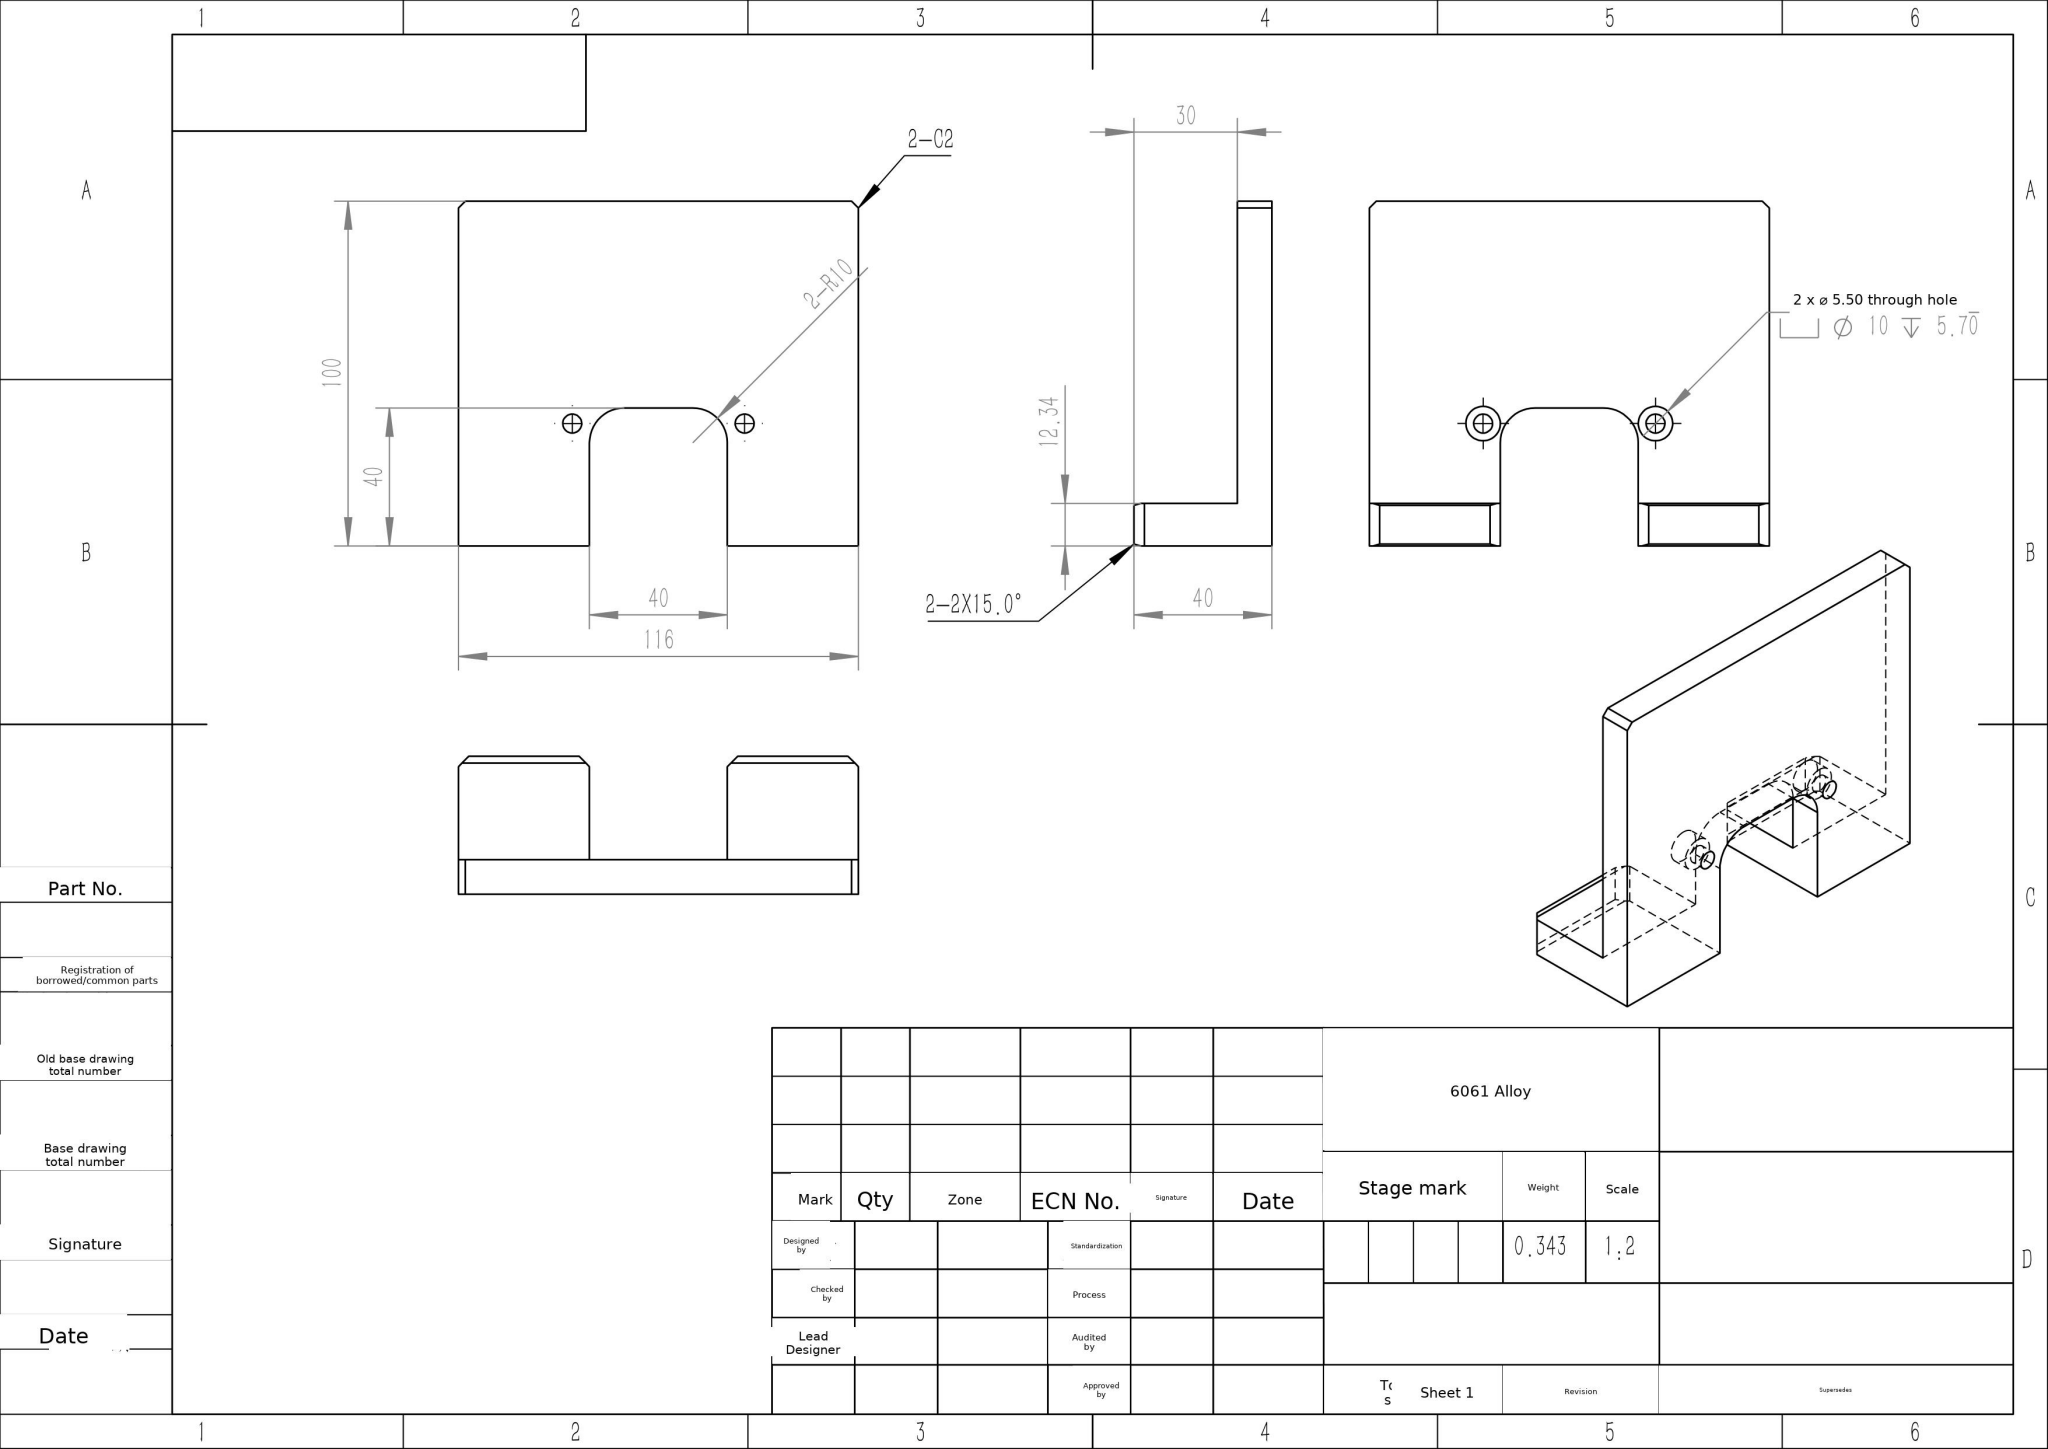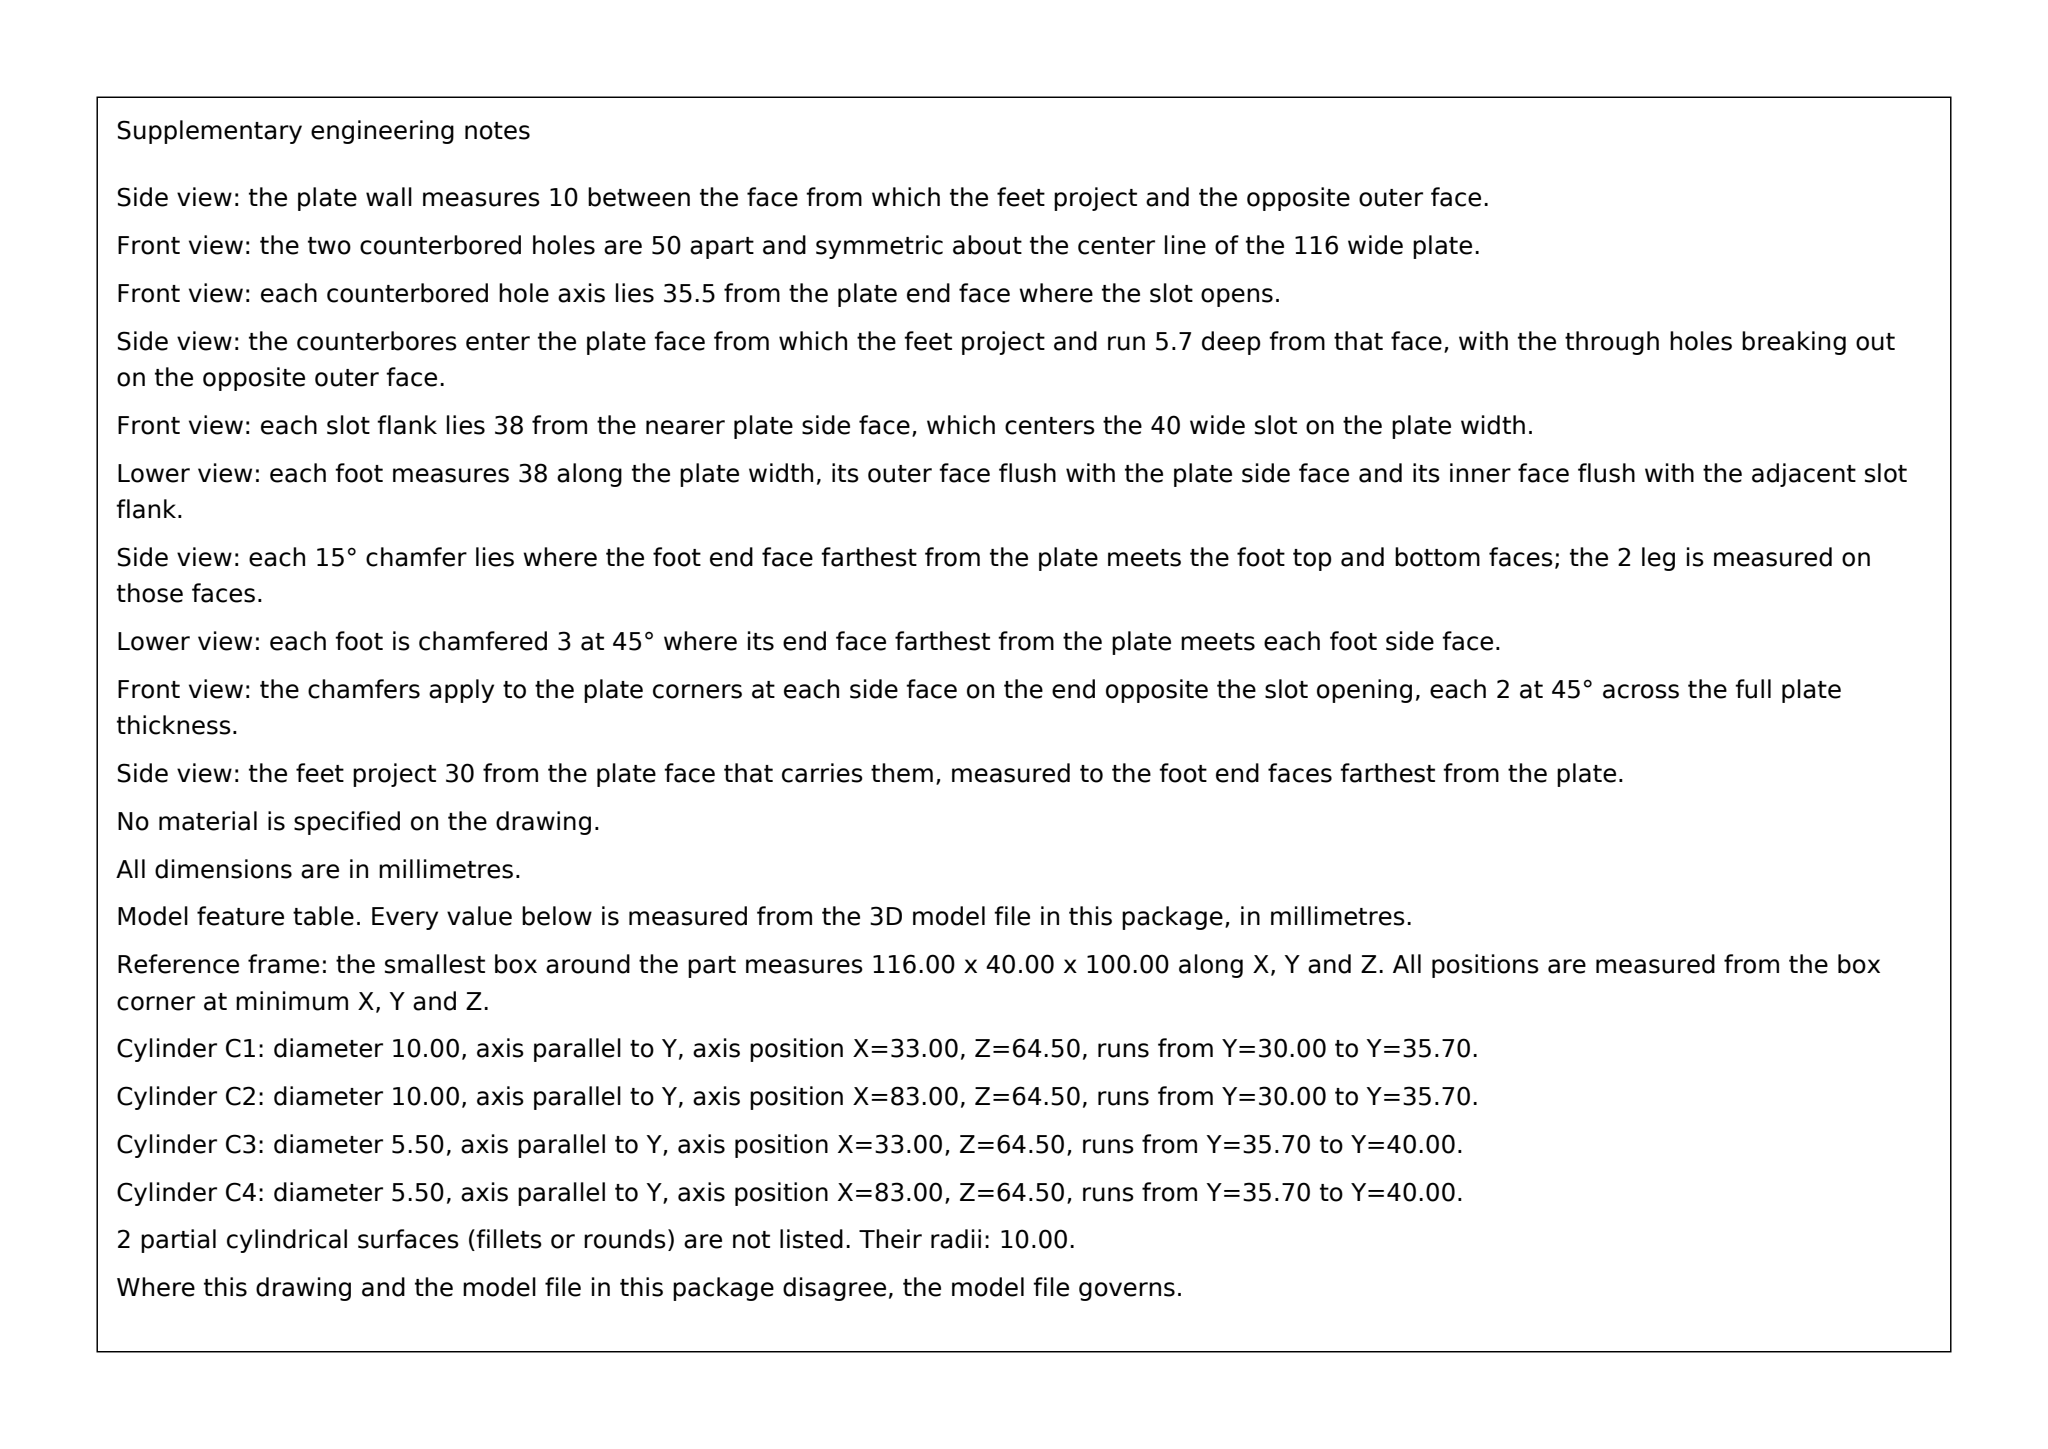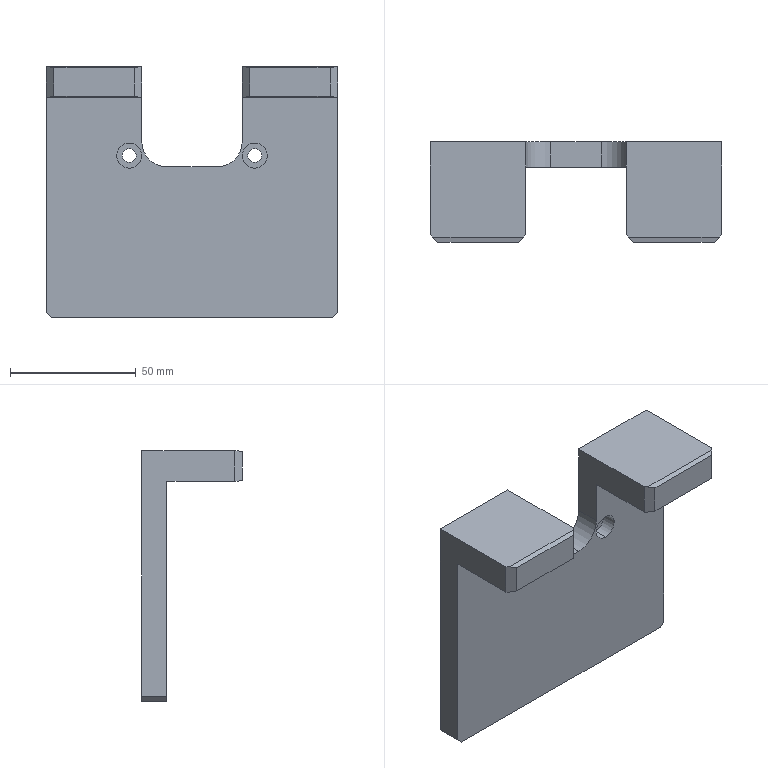Part | SolidWorks | mm | 1 solid | 36 faces | box 116 x 40 x 100 mm | volume 127128 mm3 | plane 26 | cylinder 10 | commonest cylinder face diameters 10 x4 5.5 x4 20 x2
Drawing notes:
2X Ø5.50 CBORE HOLES: 33 & 83 FROM LH EDGE, 50 CTR-CTR | from the solid: cyl dia5.5/dia10 at x=33.0 and x=83.0 (bbox x=116, so symm abt CL; spacing 50)
CBORE HOLE CL 64.5 FROM TOP EDGE (35.5 FROM BOT EDGE) | from the solid: cyl pos z=64.5 of 100 tall bbox; slot top plane z=60 = 40 from bottom
VERT PLATE THK 10 (SIDE VIEW FACES 30 TO 40) | from the solid: y-normal planes at 30.0 and 40.0; bbox y=40
2-2X15.0° CHAMF ON FRONT BOT EDGE OF EA FOOT, BASE THK 12.34 | from the solid: z-planes 87.66 (2X, foot top) vs bbox z=100; chamfer edge at y=0 / z=100
build123d program:
from build123d import *
from OCP.BRepFilletAPI import BRepFilletAPI_MakeChamfer

# Parameters (mm, degrees)
SKETCH1_W                                       = 116
SKETCH1_H                                       = 100
BOSS_EXTRUDE1_DEPTH                             = 10
M5_HEX_SOCKET_HEAD_CAP_SCREW_CBORE1_D           = 5.5
M5_HEX_SOCKET_HEAD_CAP_SCREW_CBORE1_DEPTH       = 10
M5_HEX_SOCKET_HEAD_CAP_SCREW_CBORE1_CBORE_D     = 10
M5_HEX_SOCKET_HEAD_CAP_SCREW_CBORE1_CBORE_DEPTH = 5.7
F_5_0MM_DOWEL_PIN_HOLE1_D                       = 5
F_5_0MM_DOWEL_PIN_HOLE1_DEPTH                   = 10
F_12_0_12_DIAMETER_HOLE1_D                      = 12
CHAMFER1_SIZE                                   = 2
CUT_EXTRUDE2_DEPTH                              = 78.227
SKETCH10_W                                      = 38
SKETCH10_H                                      = 12.339
BOSS_EXTRUDE2_DEPTH                             = 30
CHAMFER2_SIZE                                   = 2
CHAMFER2_SIZE2                                  = 0.5359
CHAMFER3_SIZE                                   = 3


with BuildPart() as part:
    # Sketch1 → Boss-Extrude1 (new body)
    with BuildSketch(Plane(origin=(0, 0, 0), x_dir=(1, 0, 0), z_dir=(0, 1, 0))):
        Rectangle(SKETCH1_W, SKETCH1_H)
    extrude(amount=BOSS_EXTRUDE1_DEPTH)

    # M5 Hex Socket Head Cap Screw CBORE1
    with Locations(Plane(origin=(0, 0, 0), x_dir=(-1, 0, 0), z_dir=(0, -1, 0))):
        with Locations((-25, 55.5), (25, 55.5), (25, -14.5), (-25, -14.5)):
            CounterBoreHole(M5_HEX_SOCKET_HEAD_CAP_SCREW_CBORE1_D / 2, M5_HEX_SOCKET_HEAD_CAP_SCREW_CBORE1_CBORE_D / 2, M5_HEX_SOCKET_HEAD_CAP_SCREW_CBORE1_CBORE_DEPTH, depth=M5_HEX_SOCKET_HEAD_CAP_SCREW_CBORE1_DEPTH)

    # 5.0mm Dowel Pin Hole1
    with Locations(Plane(origin=(0, 0, 0), x_dir=(-1, 0, 0), z_dir=(0, -1, 0))):
        with Locations((15, 55.5), (-15, -14.5)):
            Hole(F_5_0MM_DOWEL_PIN_HOLE1_D / 2, depth=F_5_0MM_DOWEL_PIN_HOLE1_DEPTH)

    # 12.0 _12_ Diameter Hole1 (through all)
    with Locations(Plane(origin=(0, 0, 0), x_dir=(-1, 0, 0), z_dir=(0, -1, 0))):
        with Locations((10, -47.5)):
            Hole(F_12_0_12_DIAMETER_HOLE1_D / 2)

    # Chamfer1
    chamfer1_edges = [part.edges().sort_by_distance(p)[0] for p in [
        (-58, 5, -50),
        (58, 5, -50),
    ]]
    chamfer(chamfer1_edges, length=CHAMFER1_SIZE)

    # Sketch9 → Cut-Extrude2 (cut, through all)
    with BuildSketch(Plane.XZ):
        with BuildLine():
            Line((20, 50), (20, 48))
            Line((20, 48), (20, 20))
            ThreePointArc((20, 20), (17.071, 12.929), (10, 10))
            Line((10, 10), (-10, 10))
            ThreePointArc((-10, 10), (-17.071, 12.929), (-20, 20))
            Line((-20, 20), (-20, 50))
            Line((-20, 50), (20, 50))
        make_face()
    extrude(amount=-CUT_EXTRUDE2_DEPTH, mode=Mode.SUBTRACT)

    # Sketch10 → Boss-Extrude2 (add)
    with BuildSketch(Plane.XZ):
        with Locations((39, 43.831)):
            Rectangle(SKETCH10_W, SKETCH10_H)
        with Locations((-39, 43.831)):
            Rectangle(SKETCH10_W, SKETCH10_H)
    extrude(amount=BOSS_EXTRUDE2_DEPTH)

    # Chamfer2: one chamfer whose edges measure the first distance from different faces: ONE call of the kernel's chamfer builder (chamfer() names one face for all edges)
    chamfer2_edges_1 = [part.edges().sort_by_distance(p)[0] for p in [
        (-39, -30, 37.661),
    ]]
    chamfer2_side_1 = [part.faces().sort_by_distance(p)[0] for p in [
        (-39, -15, 37.661),
    ]]
    chamfer2_edges_2 = [part.edges().sort_by_distance(p)[0] for p in [
        (-39, -30, 50),
    ]]
    chamfer2_side_2 = [part.faces().sort_by_distance(p)[0] for p in [
        (-39, -10, 50),
    ]]
    chamfer2_edges_3 = [part.edges().sort_by_distance(p)[0] for p in [
        (39, -30, 50),
    ]]
    chamfer2_side_3 = [part.faces().sort_by_distance(p)[0] for p in [
        (39, -10, 50),
    ]]
    chamfer2_edges_4 = [part.edges().sort_by_distance(p)[0] for p in [
        (39, -30, 37.661),
    ]]
    chamfer2_side_4 = [part.faces().sort_by_distance(p)[0] for p in [
        (39, -15, 37.661),
    ]]
    chamfer2 = BRepFilletAPI_MakeChamfer(part.part.solid().wrapped)
    for e in chamfer2_edges_1:
        chamfer2.Add(CHAMFER2_SIZE, CHAMFER2_SIZE2, e.wrapped, chamfer2_side_1[0].wrapped)  # the first distance lies on this face
    for e in chamfer2_edges_2:
        chamfer2.Add(CHAMFER2_SIZE, CHAMFER2_SIZE2, e.wrapped, chamfer2_side_2[0].wrapped)  # the first distance lies on this face
    for e in chamfer2_edges_3:
        chamfer2.Add(CHAMFER2_SIZE, CHAMFER2_SIZE2, e.wrapped, chamfer2_side_3[0].wrapped)  # the first distance lies on this face
    for e in chamfer2_edges_4:
        chamfer2.Add(CHAMFER2_SIZE, CHAMFER2_SIZE2, e.wrapped, chamfer2_side_4[0].wrapped)  # the first distance lies on this face
    add(Compound.cast(chamfer2.Shape()), mode=Mode.REPLACE)

    # Chamfer3
    chamfer3_edges = [part.edges().sort_by_distance(p)[0] for p in [
        (20, -30, 43.831),
        (58, -30, 43.831),
        (-20, -30, 43.831),
        (-58, -30, 43.831),
    ]]
    chamfer(chamfer3_edges, length=CHAMFER3_SIZE)


solid = part.part